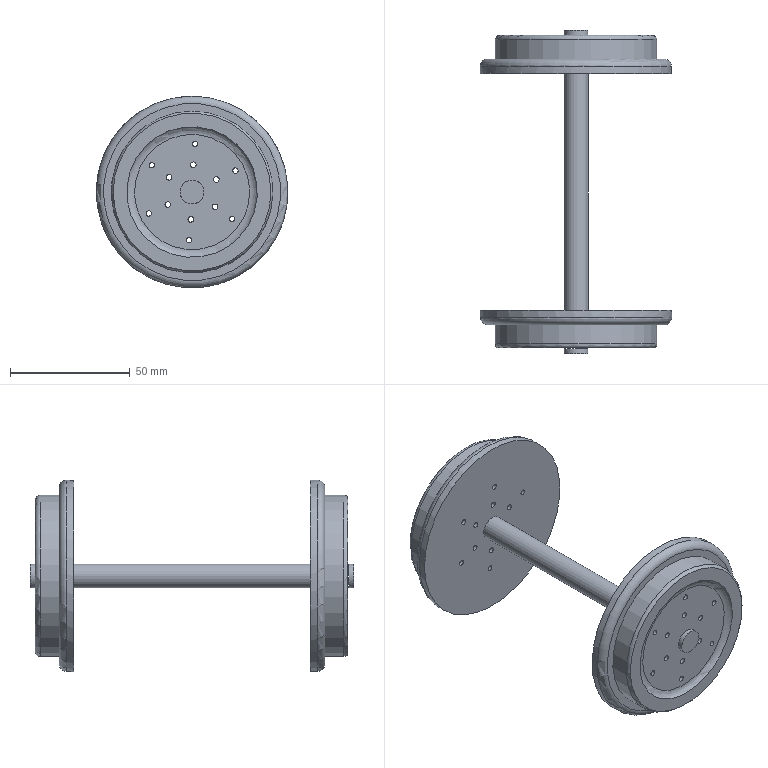Component | NX | WHEEL_HUB_3 | 2 solids | 46 faces | volume 132408 mm3 | cylinder 31 | plane 10 | torus 5 | commonest cylinder face diameters 2.235 x12 2.354 x12 10 x3 80 x2 67.525 x2